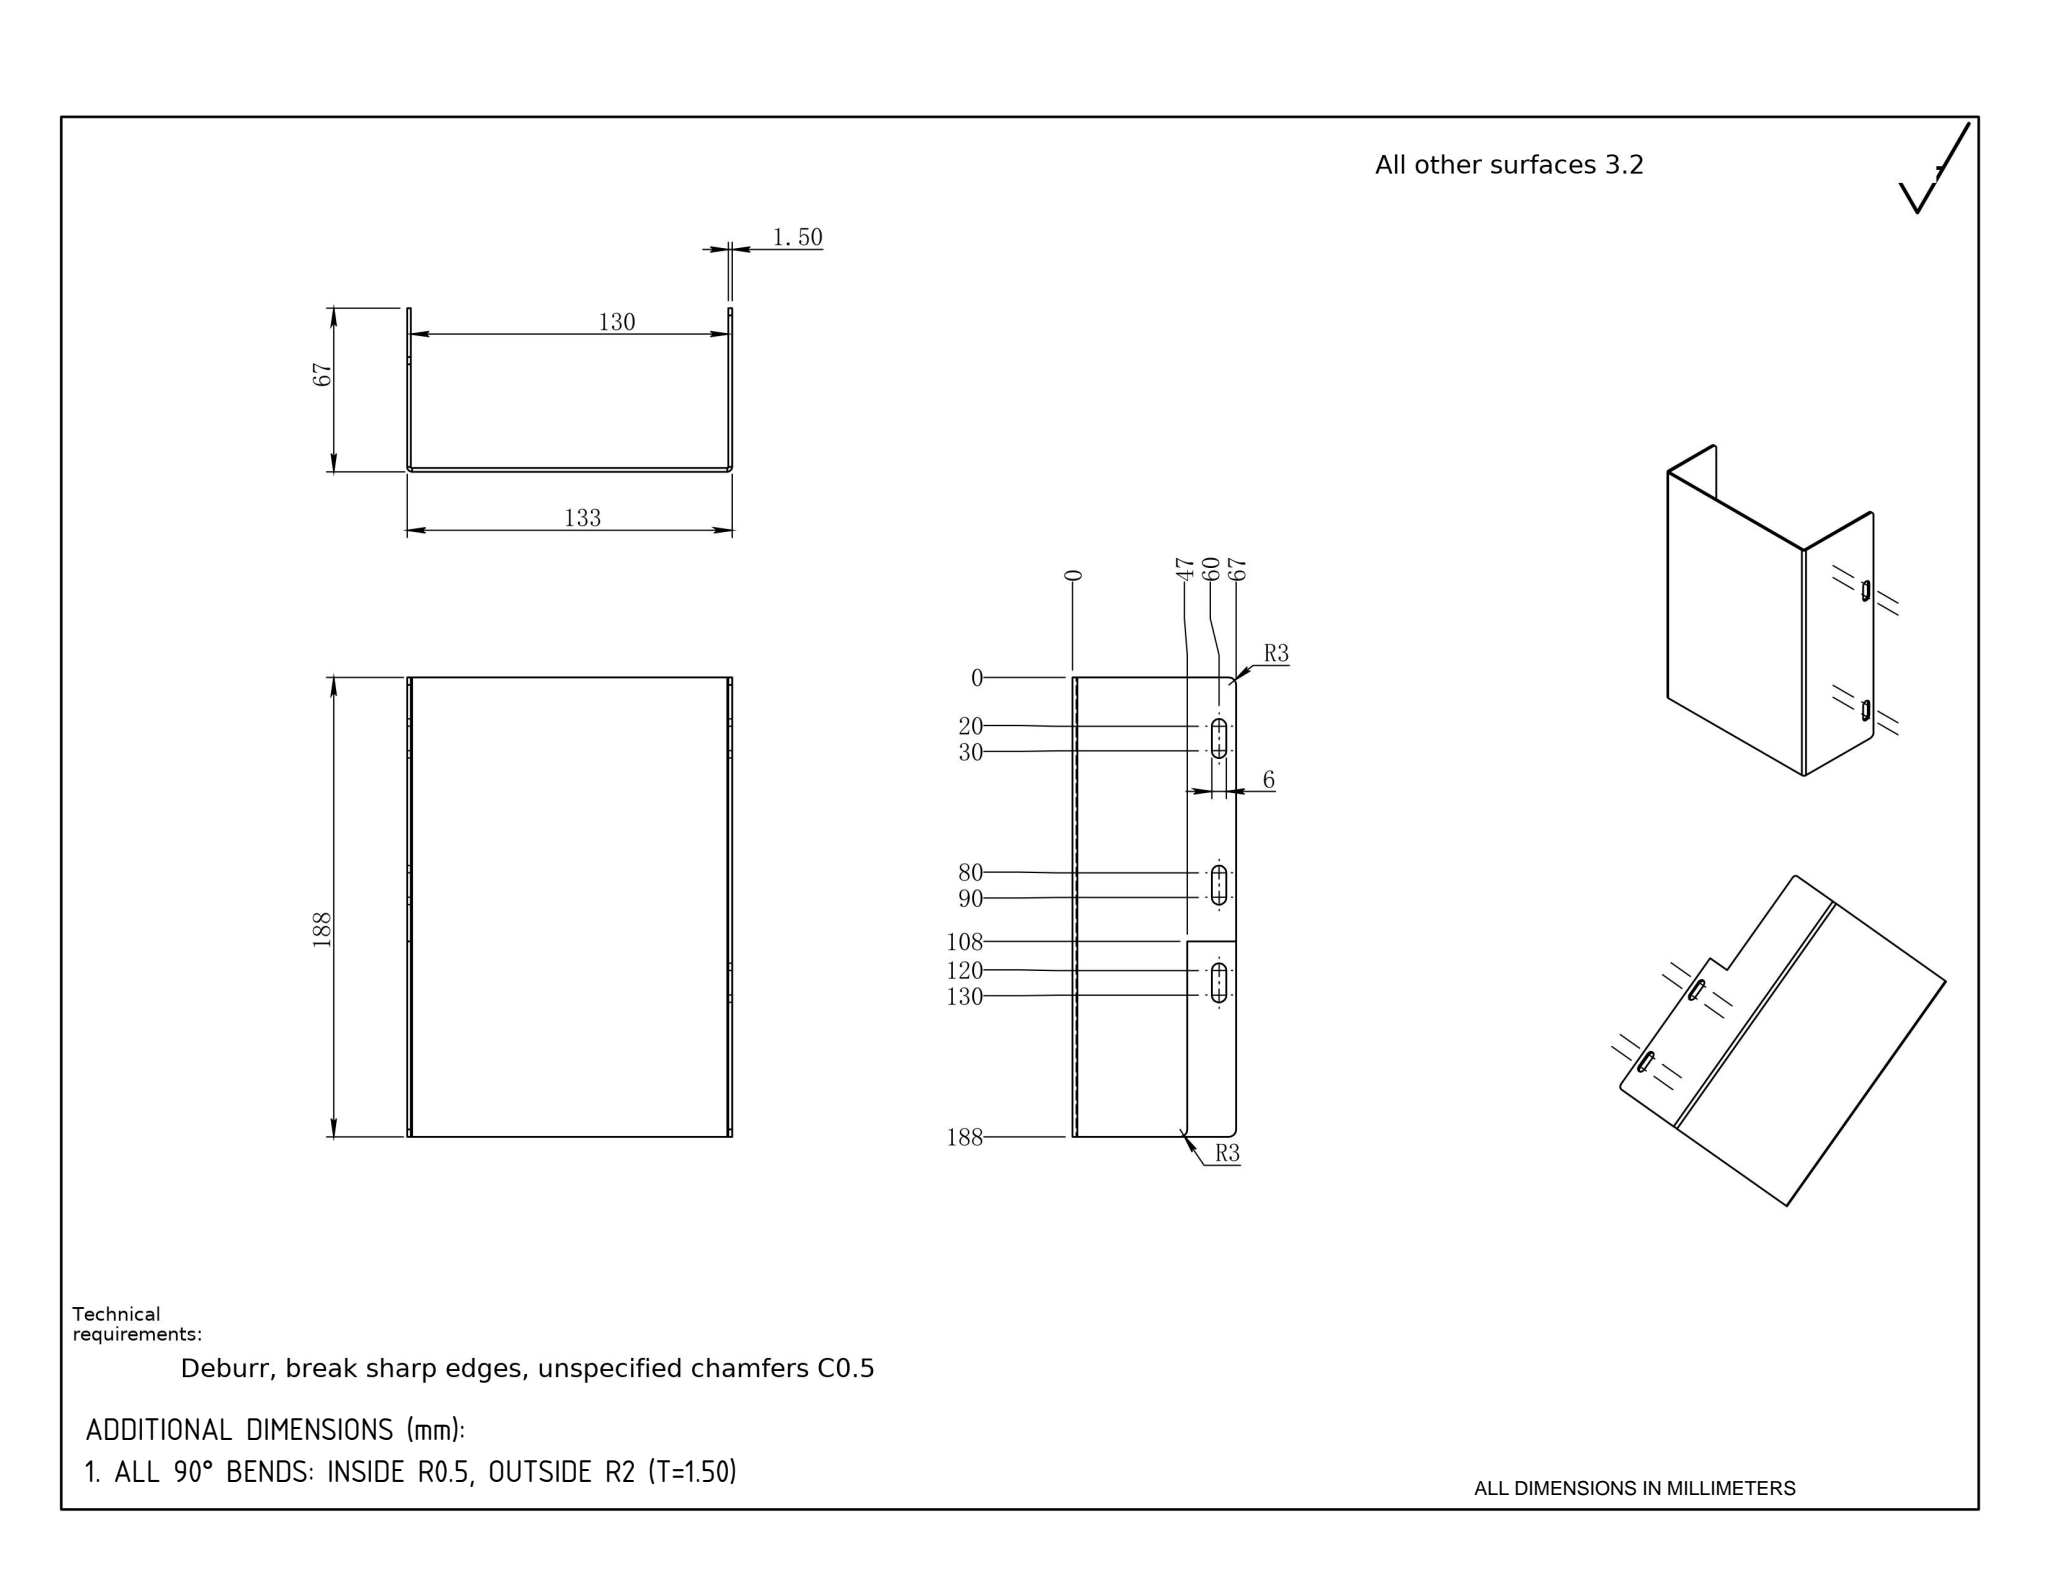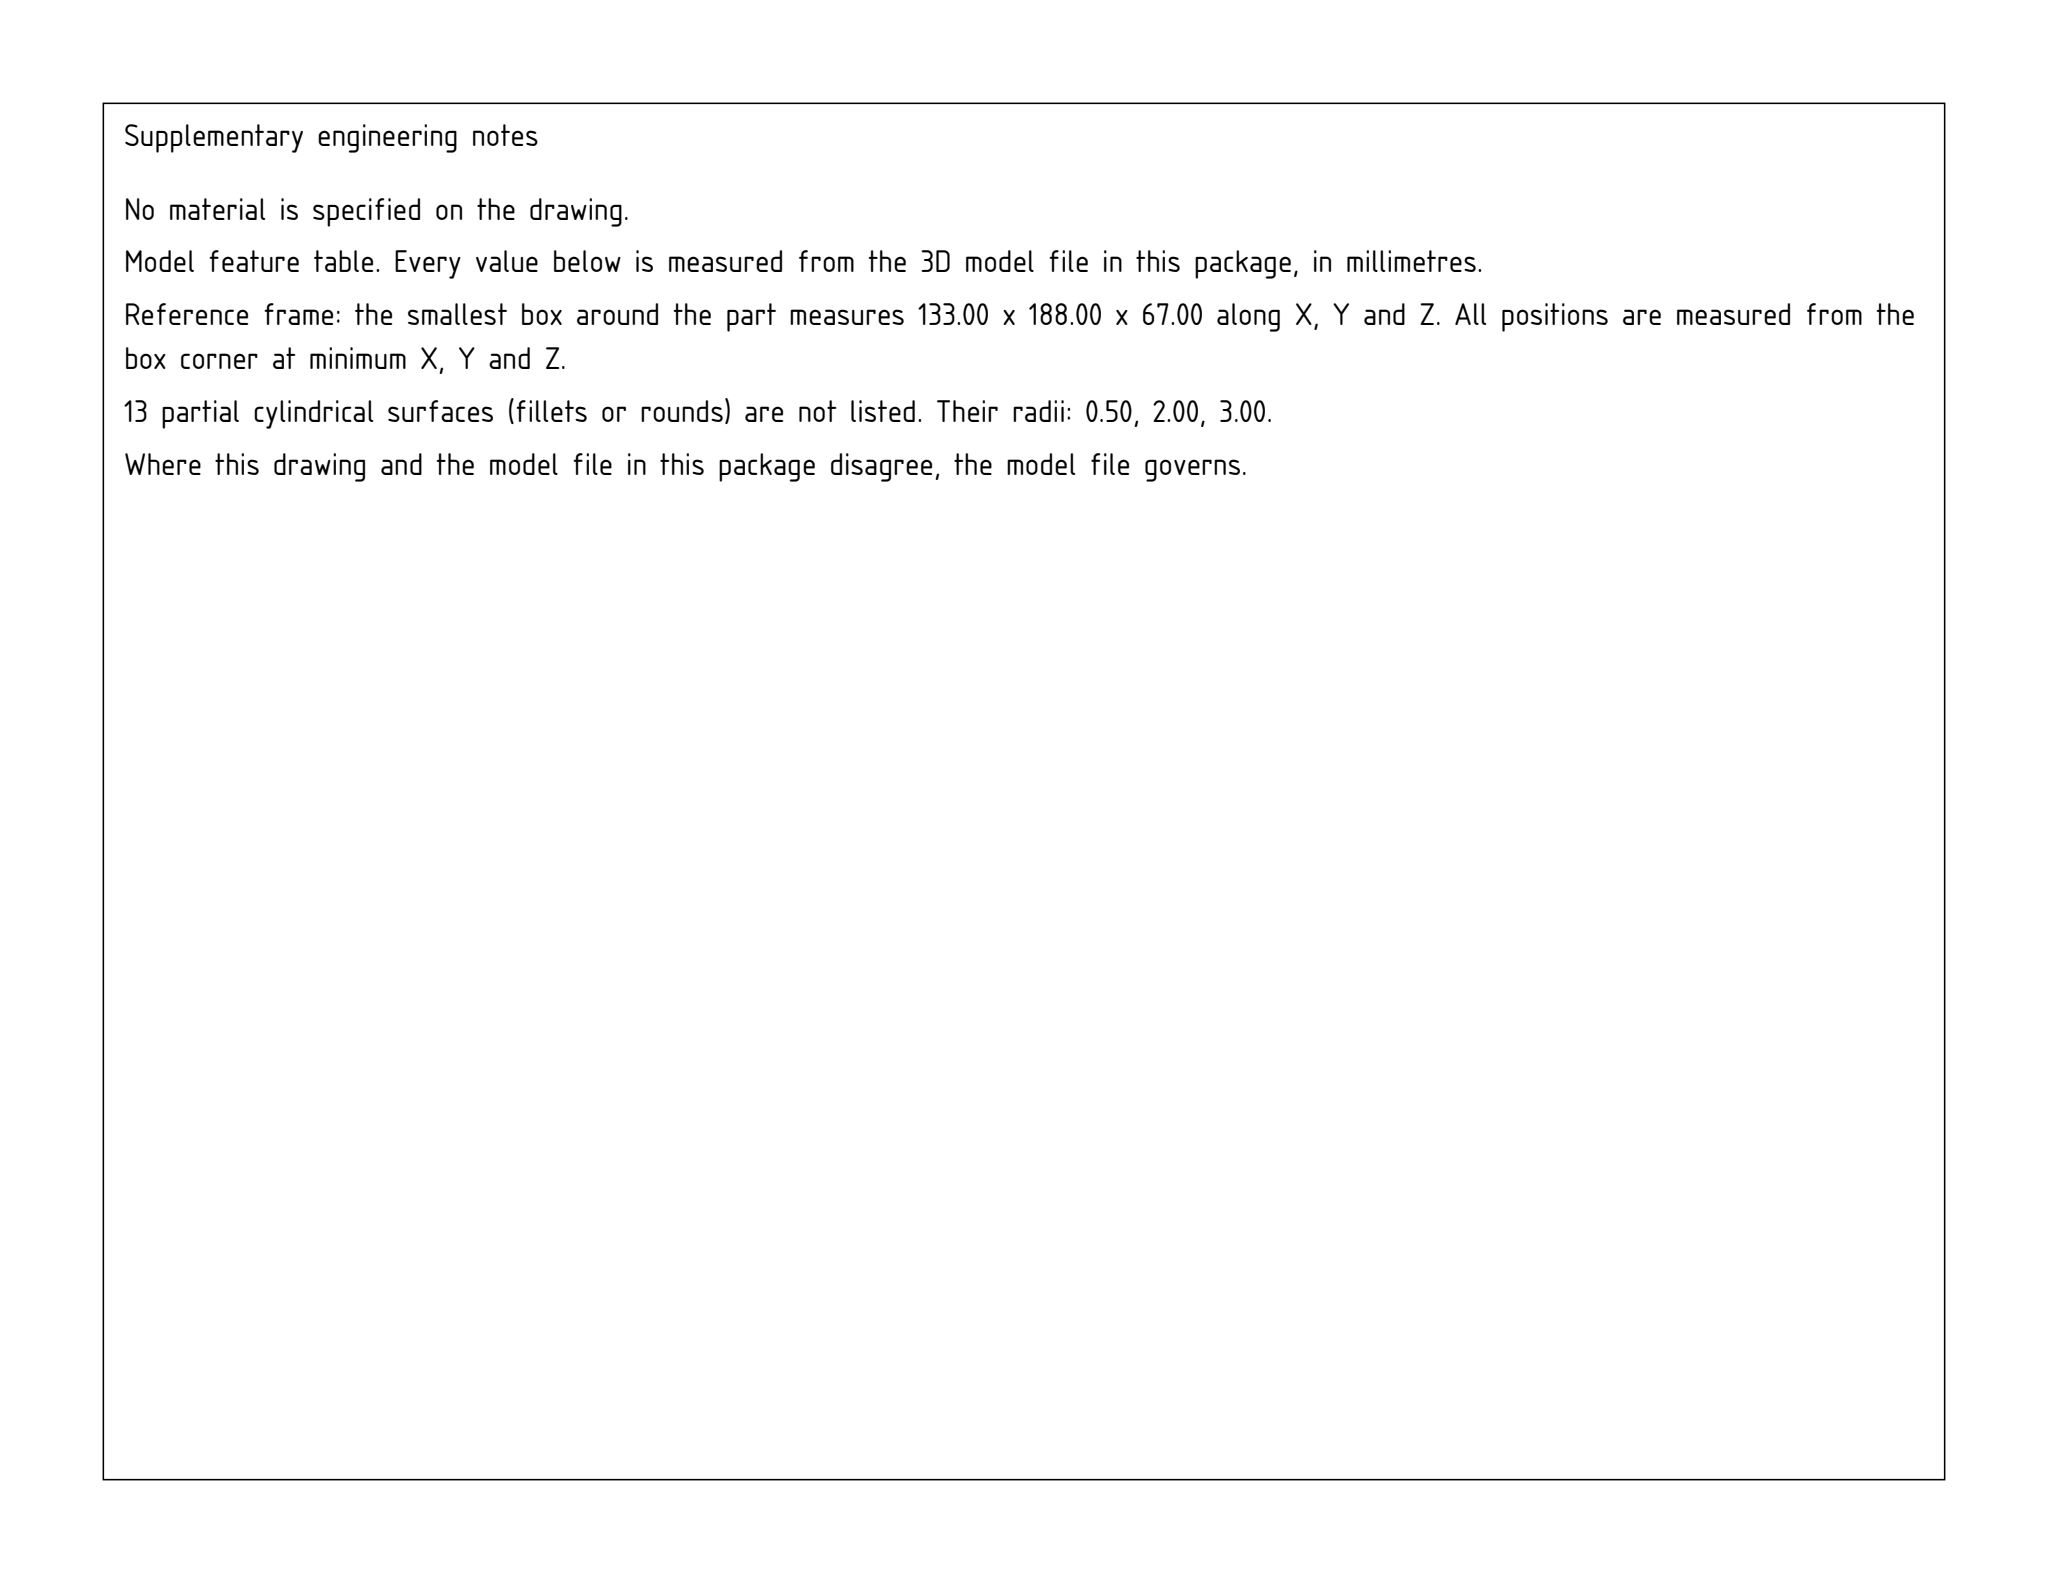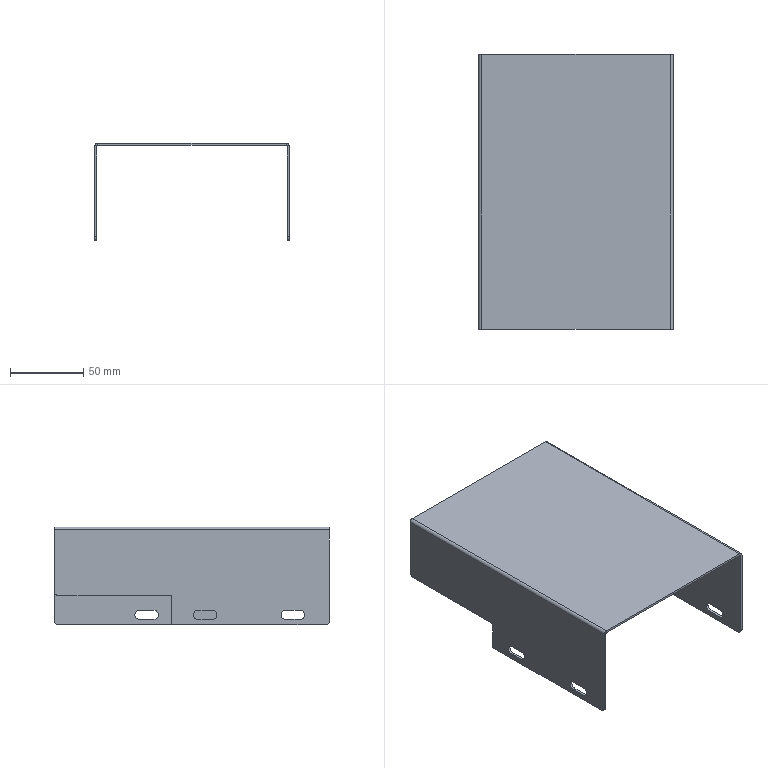Part | SolidWorks | mm | 1 solid | 44 faces | box 133 x 188 x 67 mm | volume 71204 mm3 | plane 28 | cylinder 16 | commonest cylinder face diameters 6 x12 1 x2 4 x2